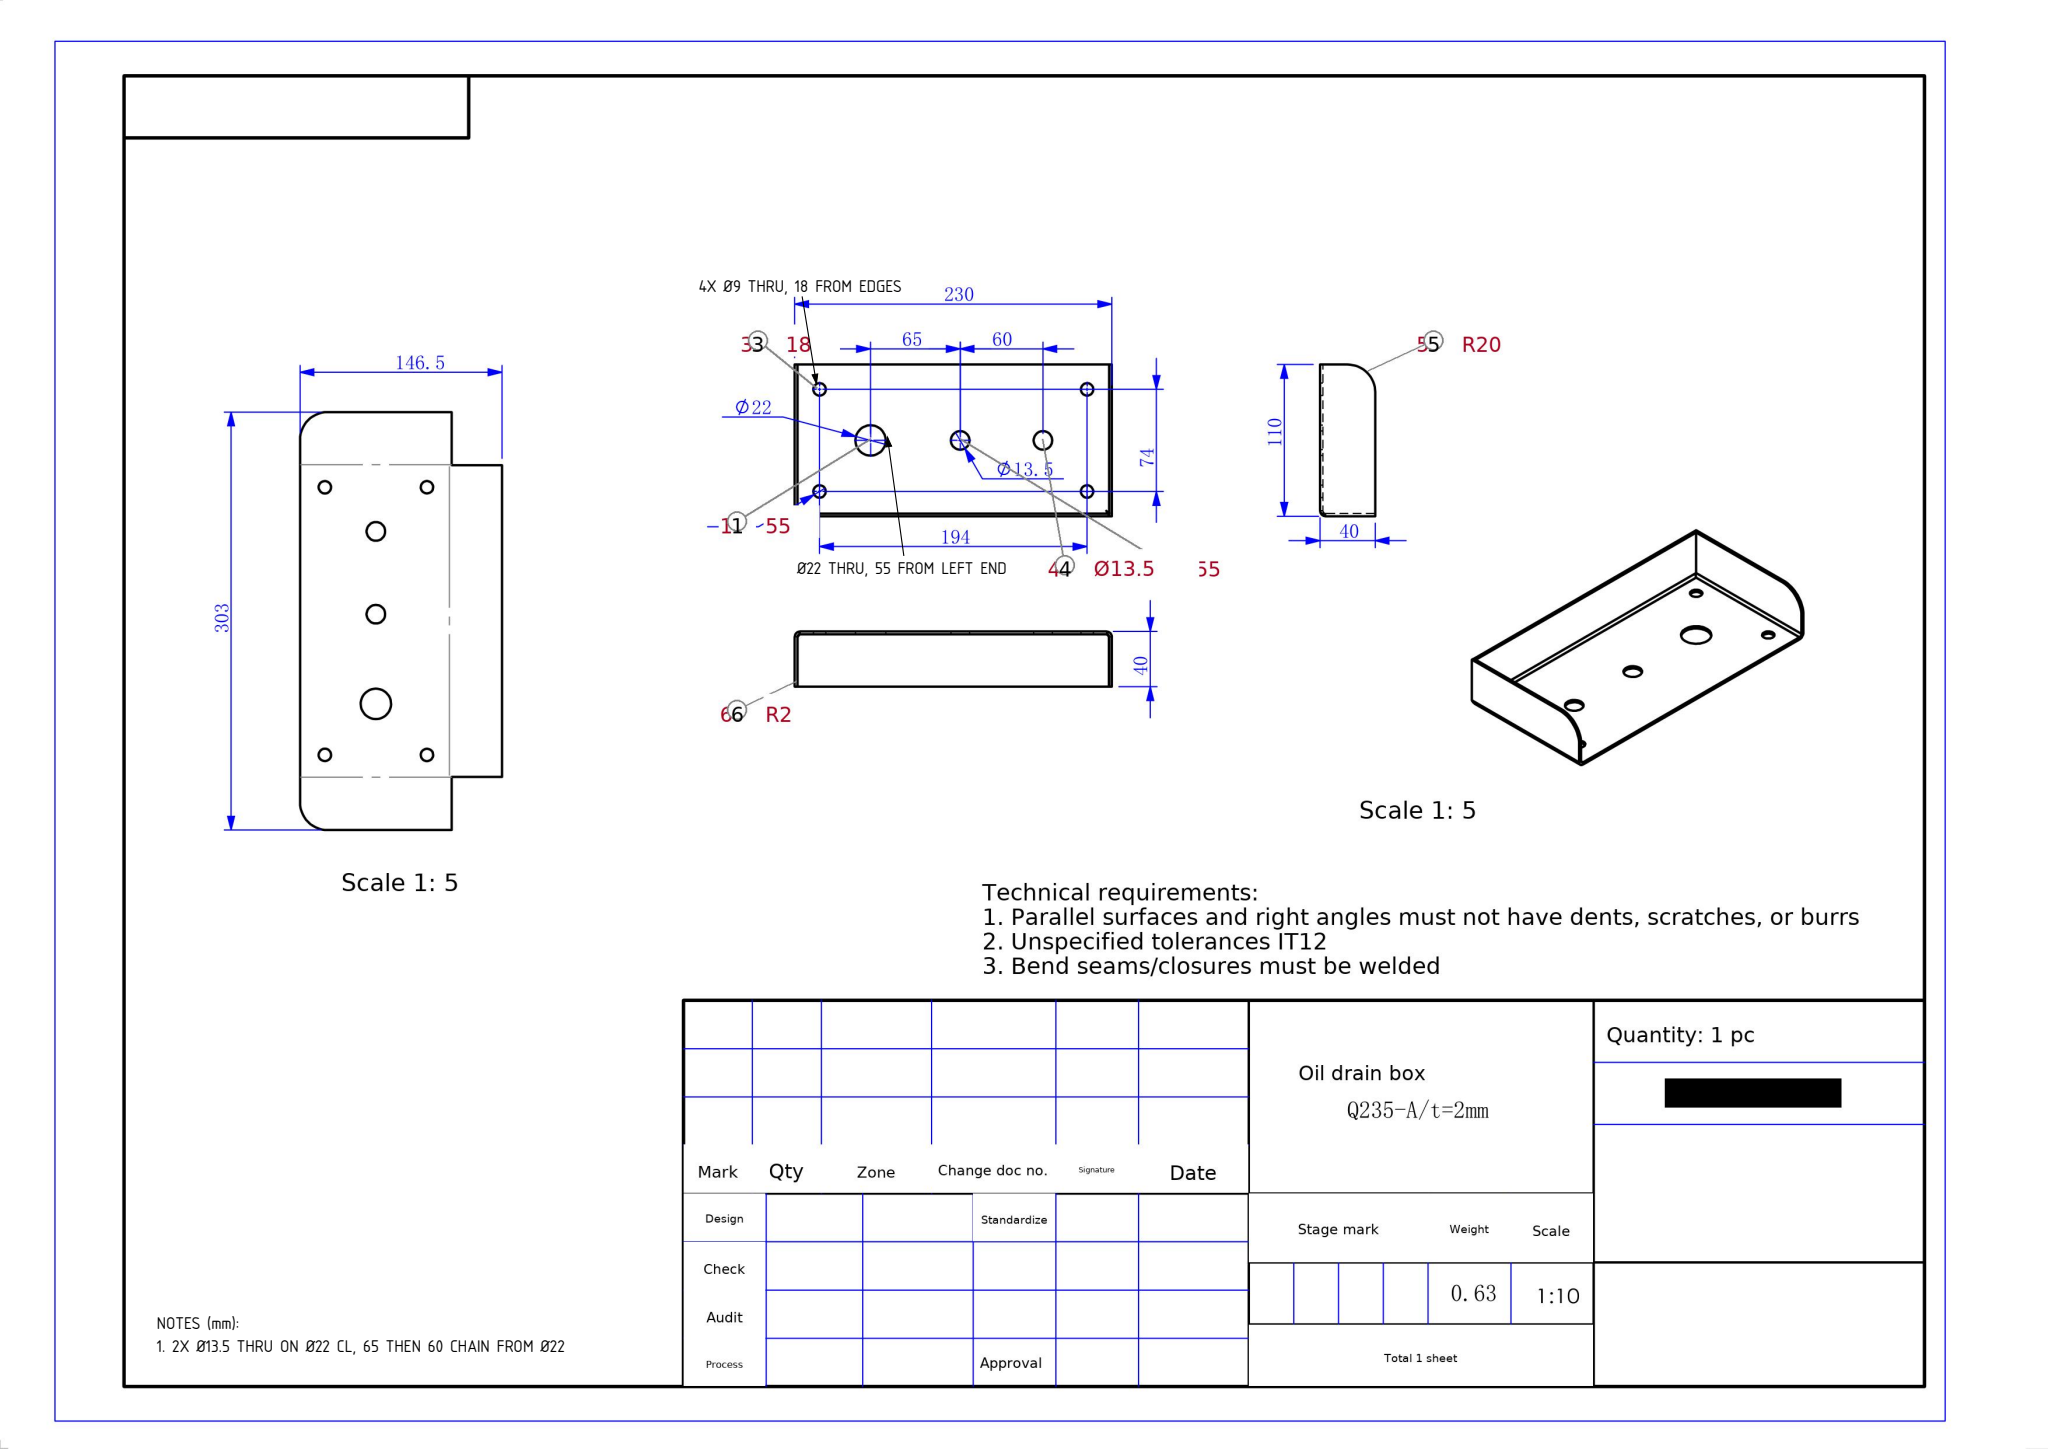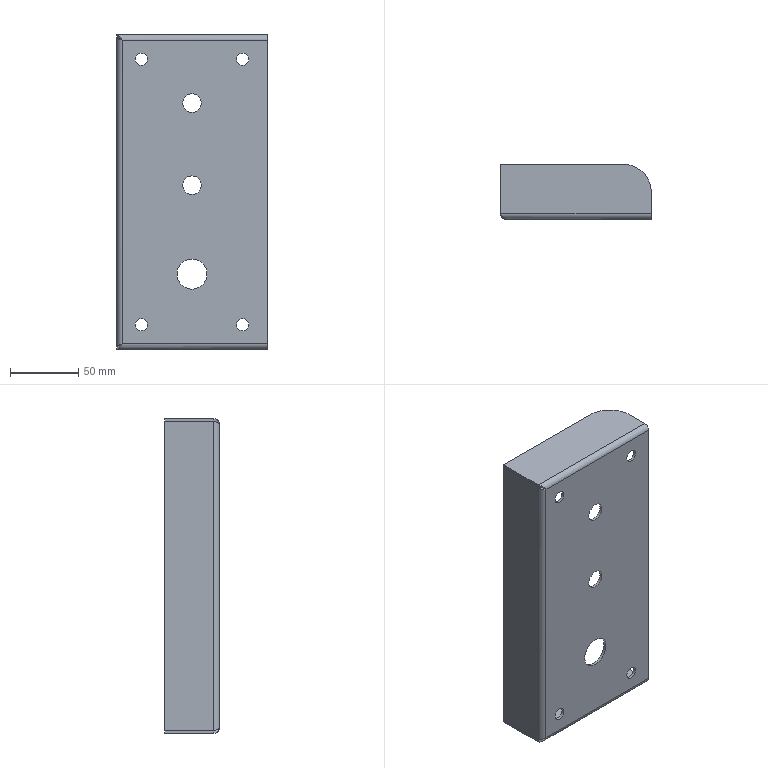Part | SolidWorks | mm | material Q235-A | 1 solid | 46 faces | box 110 x 40 x 230 mm | volume 81122 mm3 | cylinder 22 | plane 20 | spline 4 | commonest cylinder face diameters 9 x8 13.5 x4 4 x3 8 x3 22 x2 40 x2
Drawing notes:
Ø22 THRU IN BASE, CL 55 FROM LEFT END, 55 FROM SIDE EDGE | from the solid: cyl Ø22 axis y, len 2.0 at x=55.0, z=55.02; bbox 110 x 40.02 x 230.04
2X Ø13.5 THRU ON Ø22 CL, 65 THEN 60 CHAIN FROM Ø22 | from the solid: cyl Ø13.5 axis y at (55,120.02) and (55,180.02) vs Ø22 at z=55.02
4X Ø9 THRU IN BASE, 194 x 74 CL, 18 FROM EDGES | from the solid: 4 cyl Ø9 axis y len 2.0 at (18,18.02),(18,212.02),(92,18.02),(92,212.02)